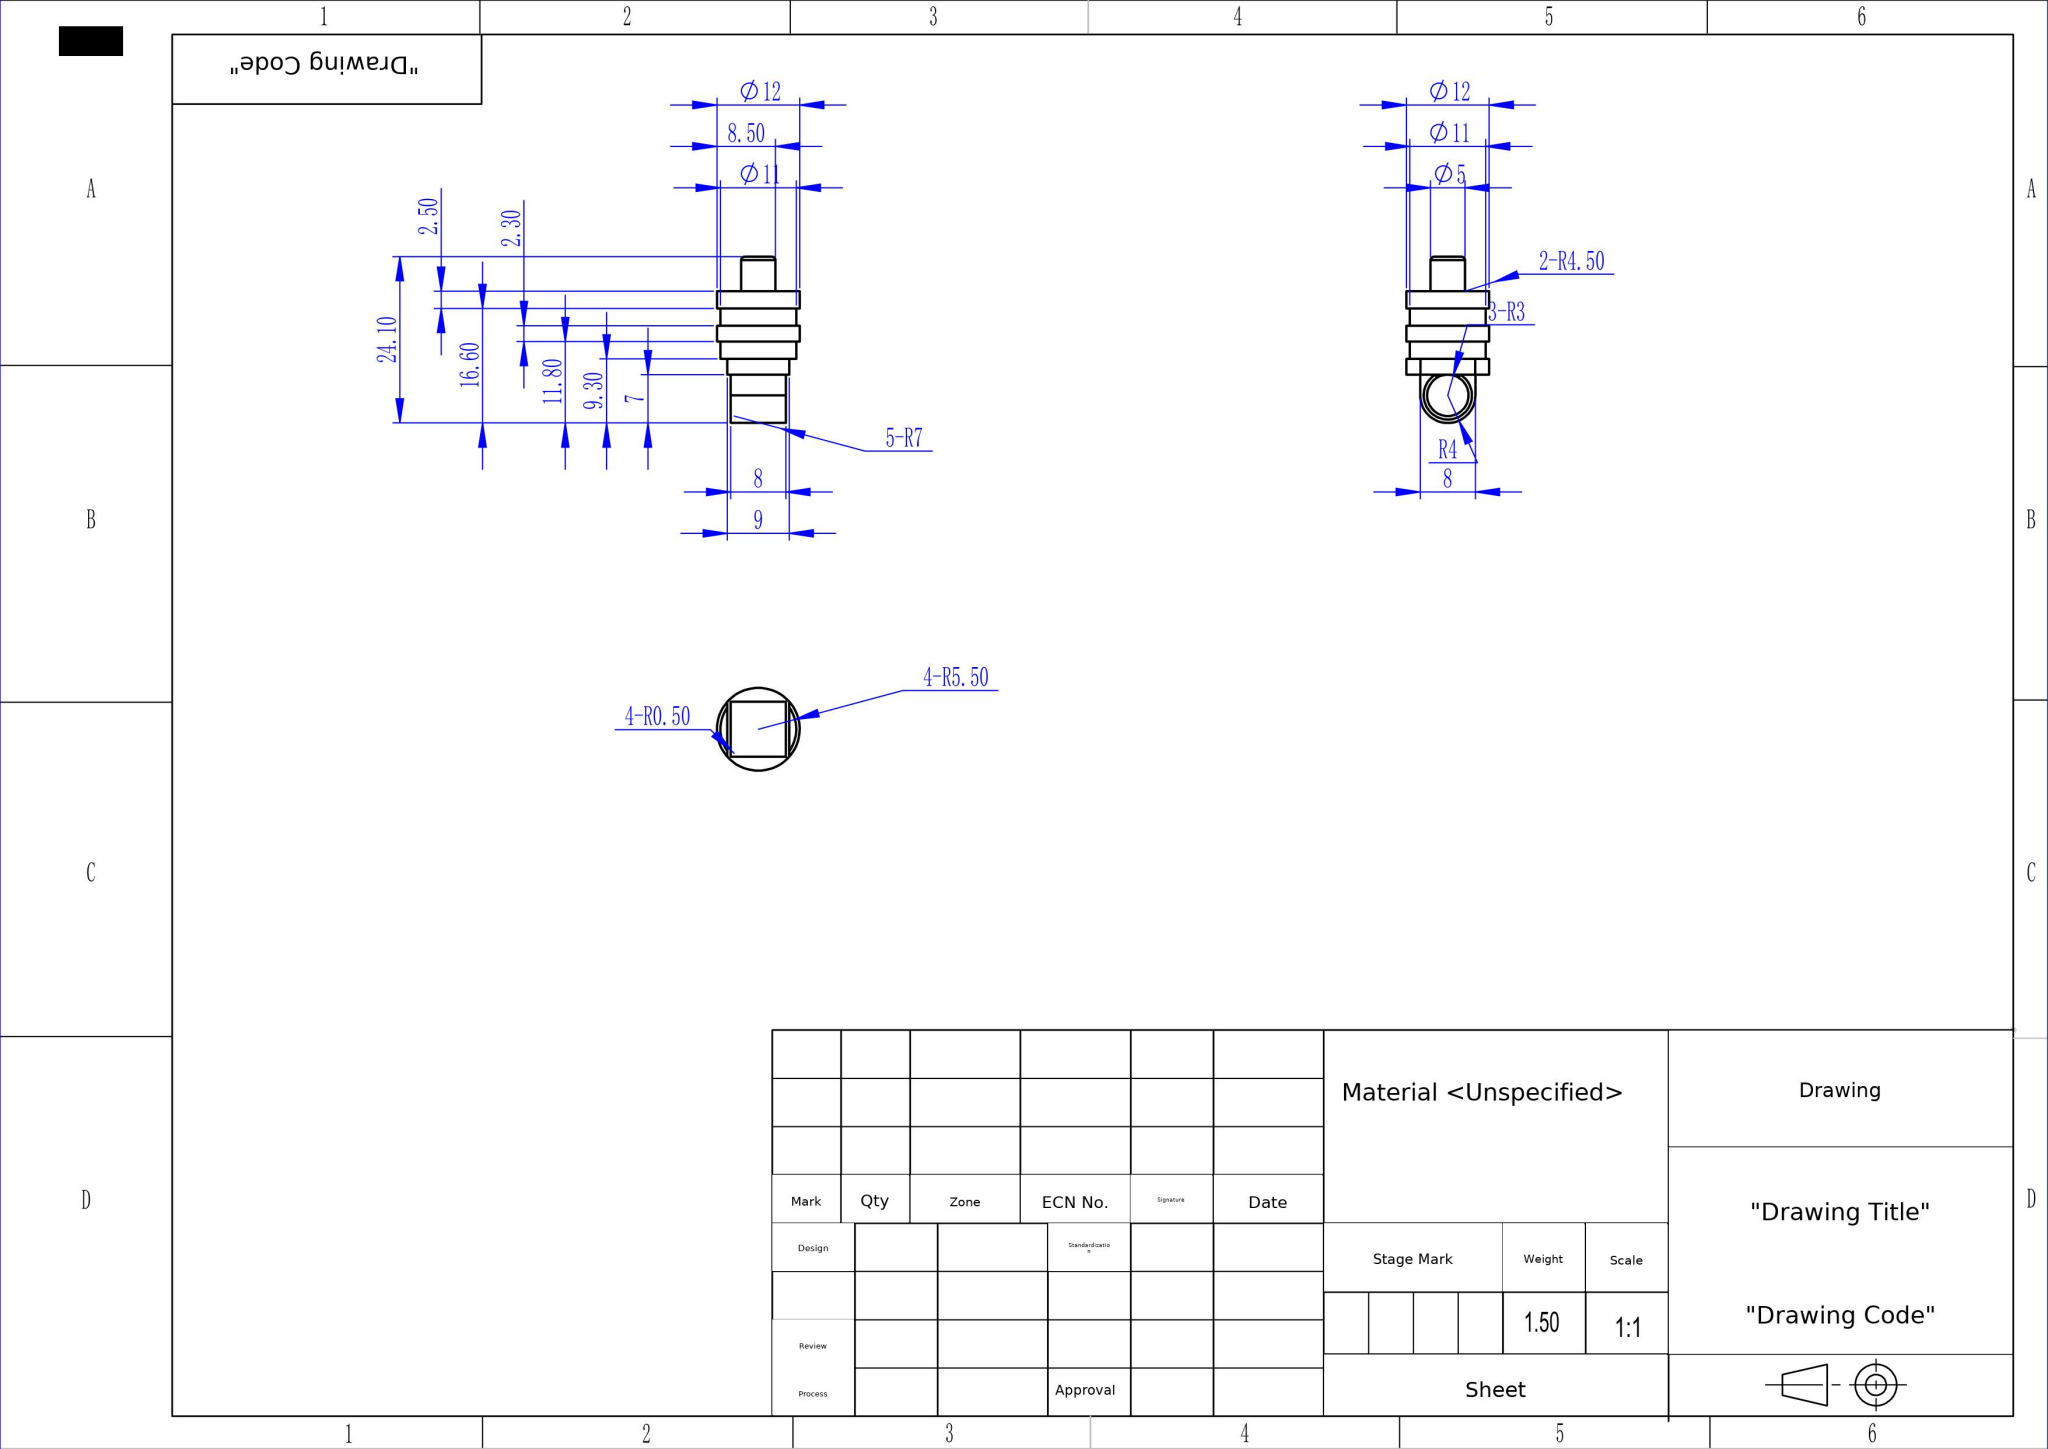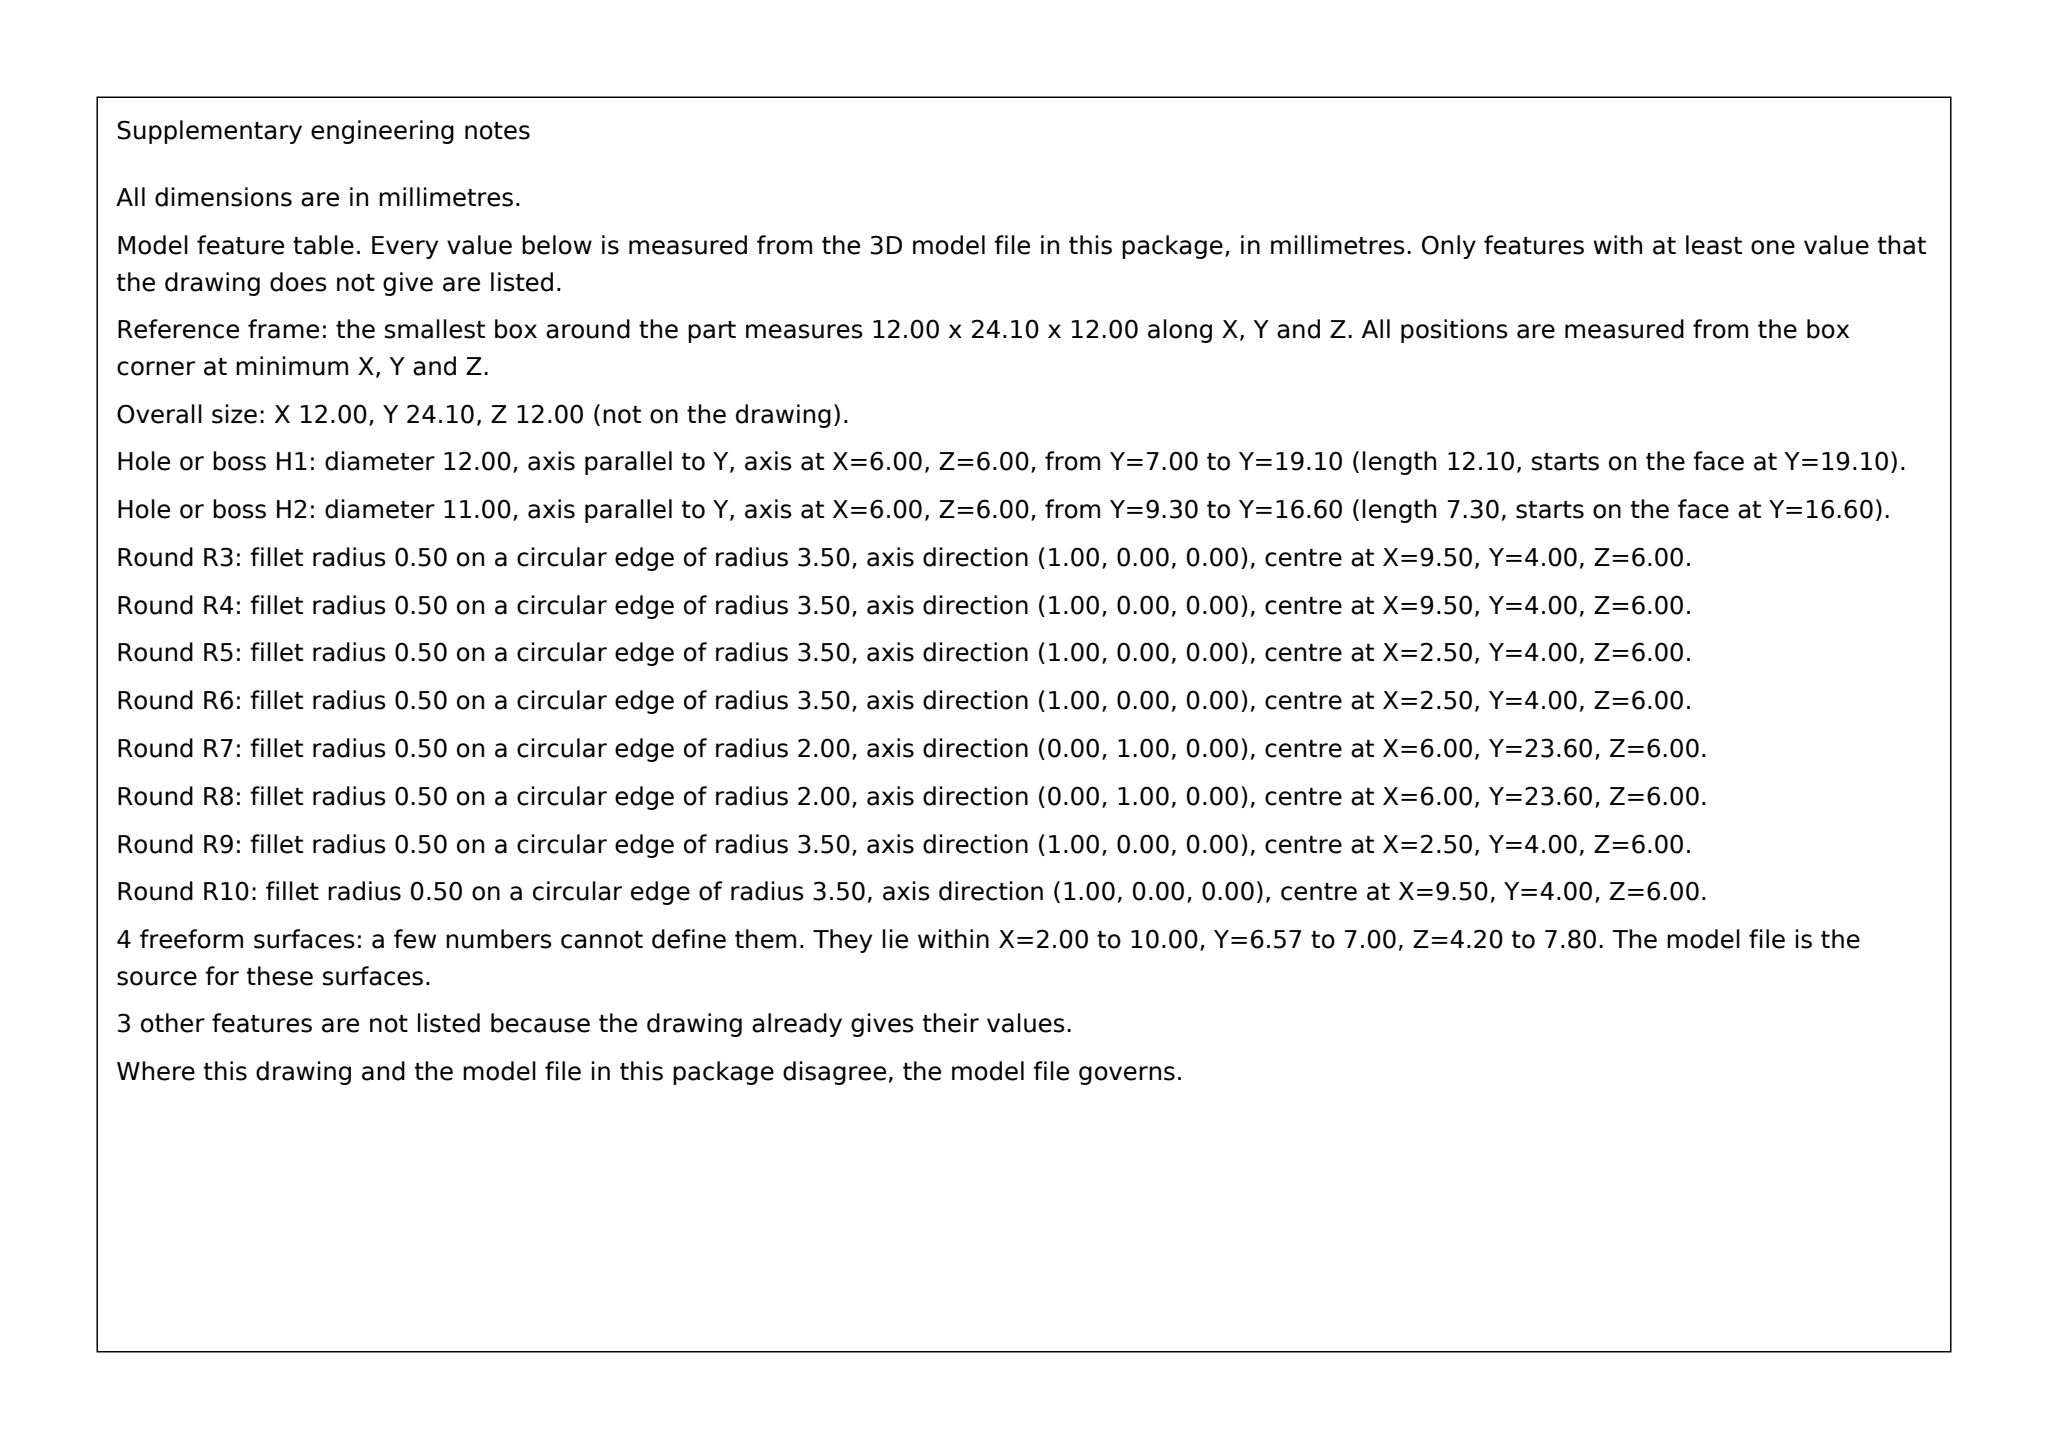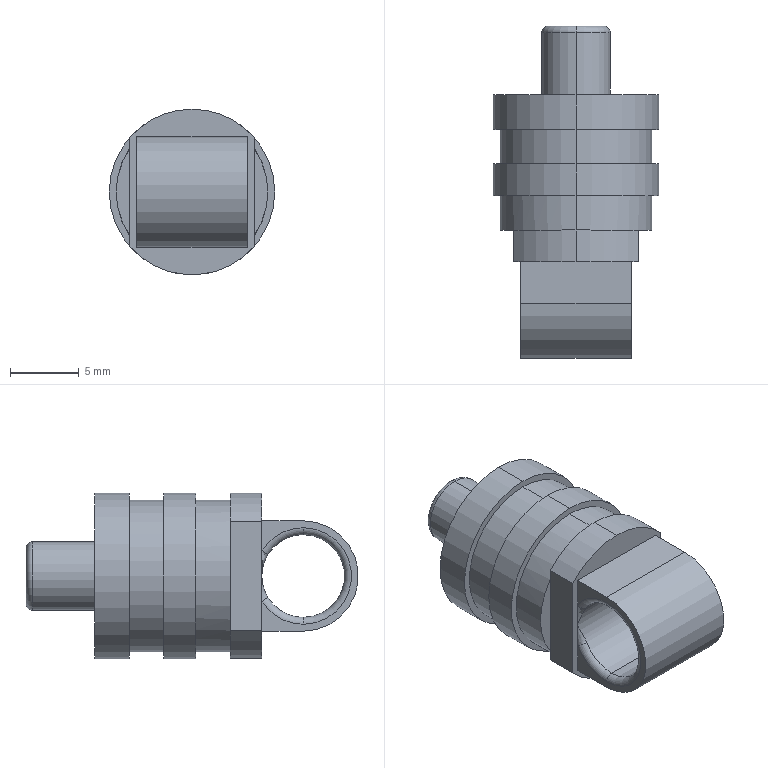Part | SolidWorks | mm | material Unspecified | 1 solid | 44 faces | box 12 x 24.1 x 12 mm | volume 1503 mm3 | cylinder 16 | plane 16 | torus 8 | spline 4 | commonest cylinder face diameters 12 x7 11 x4 6 x2 5 x2 8 x1